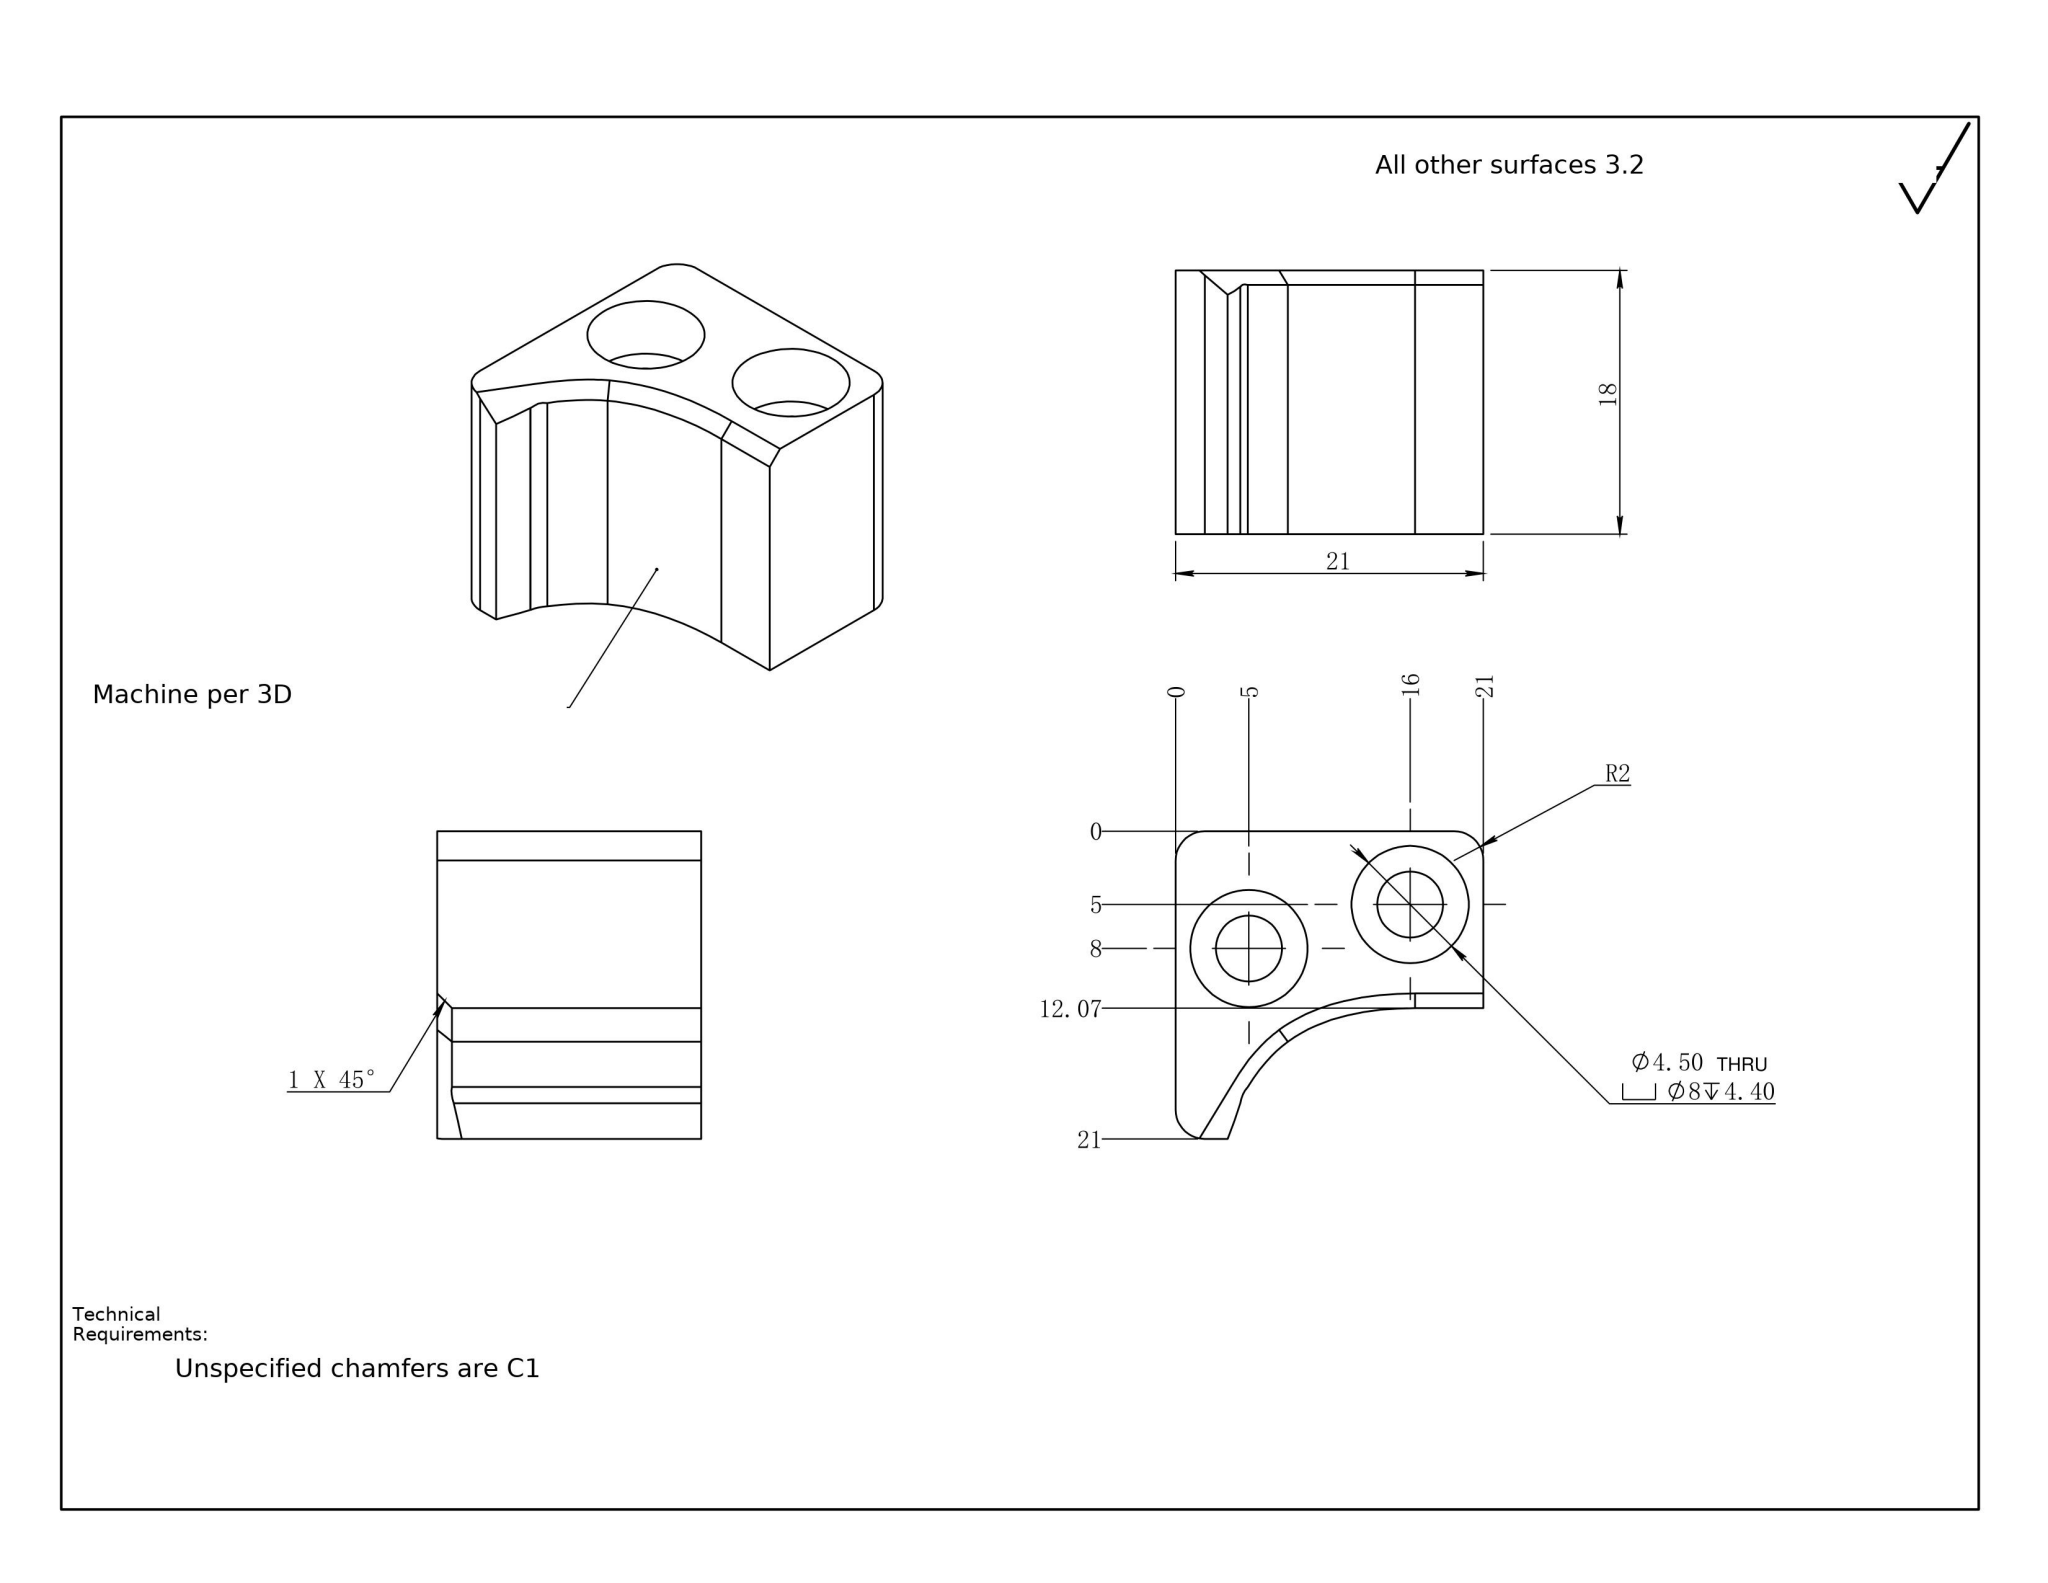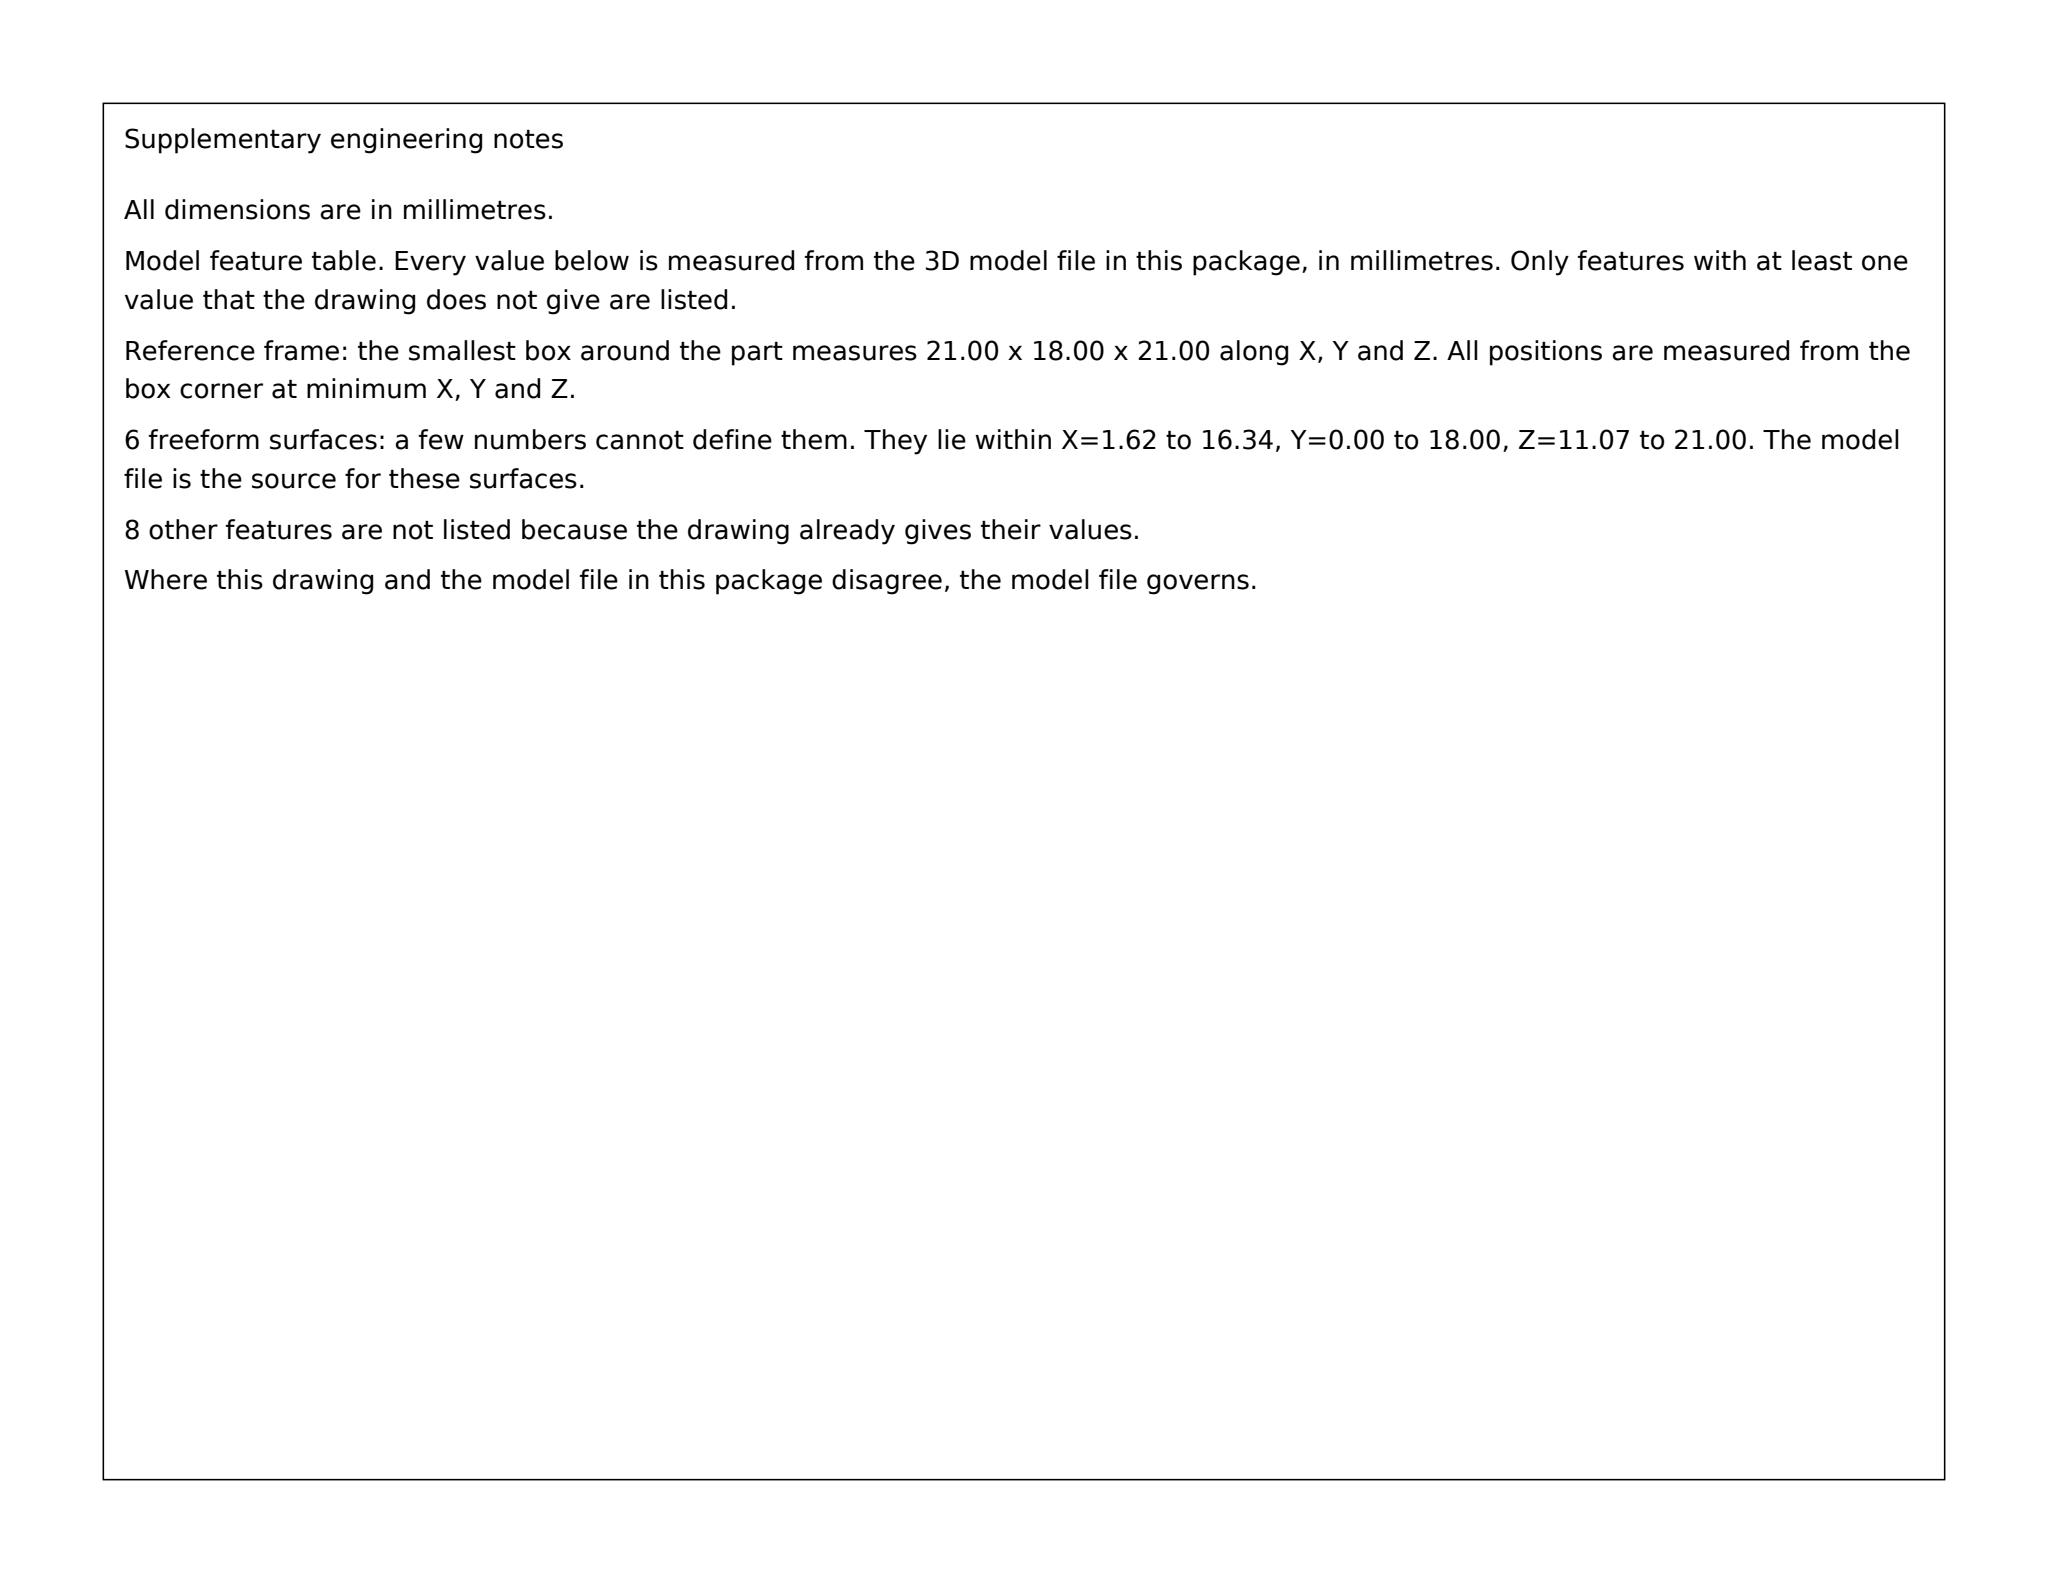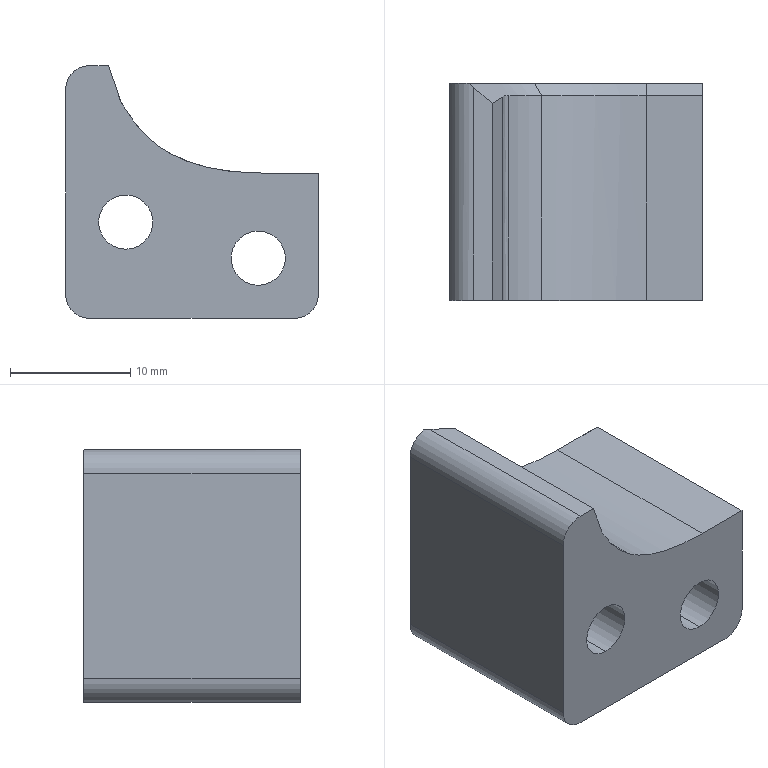Part | SolidWorks | mm | 1 solid | 28 faces | box 21 x 18 x 21 mm | volume 4654 mm3 | cylinder 11 | plane 11 | spline 6 | commonest cylinder face diameters 8 x4 4.5 x4 4 x3